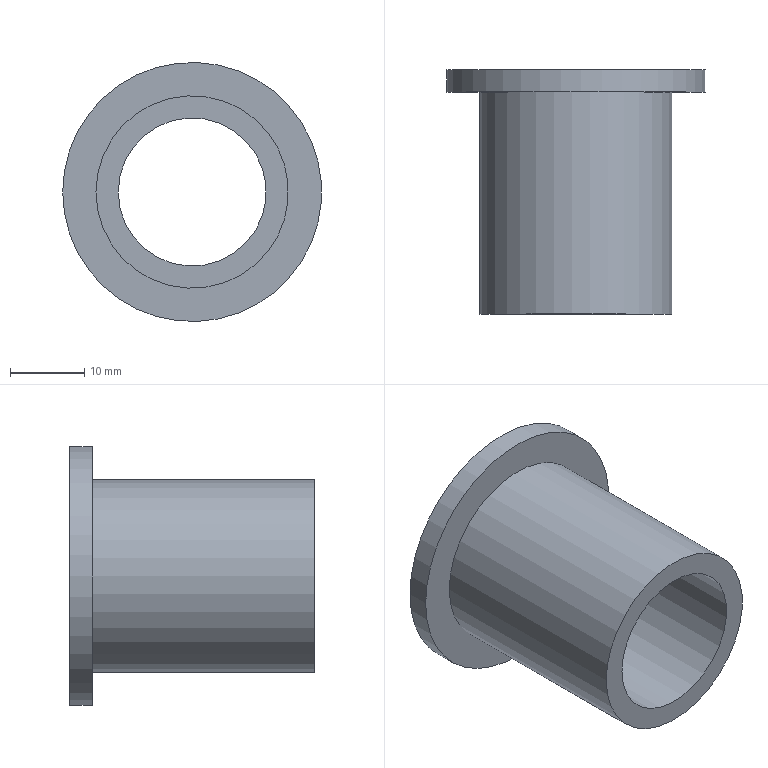Component | NX | BUSHING | 1 solid | 6 faces | box 35 x 33 x 35 mm | volume 8447 mm3 | cylinder 3 | plane 3 | commonest cylinder face diameters 26 x1 20 x1 35 x1
STEP:
#1=CARTESIAN_POINT('',(0.,0.,0.));
#2=DIRECTION('',(0.,0.,1.));
#3=DIRECTION('',(1.,0.,0.));
#4=AXIS2_PLACEMENT_3D('',#1,#2,#3);
#5=CARTESIAN_POINT('',(-13.,30.,66.));
#6=VERTEX_POINT('',#5);
#7=CARTESIAN_POINT('',(0.,30.,66.));
#8=DIRECTION('',(0.,1.,0.));
#9=DIRECTION('',(-1.,0.,0.));
#10=AXIS2_PLACEMENT_3D('',#7,#8,#9);
#11=CIRCLE('',#10,13.);
#12=CARTESIAN_POINT('',(0.,30.,66.));
#13=DIRECTION('',(0.,-1.,0.));
#14=DIRECTION('',(0.,0.,1.));
#15=AXIS2_PLACEMENT_3D('',#12,#13,#14);
#16=CYLINDRICAL_SURFACE('',#15,13.);
#17=CARTESIAN_POINT('',(7.854,0.));
#18=DIRECTION('',(-1.,0.));
#19=VECTOR('',#18,1.);
#20=LINE('',#17,#19);
#21=(GEOMETRIC_REPRESENTATION_CONTEXT(2)PARAMETRIC_REPRESENTATION_CONTEXT()REPRESENTATION_CONTEXT('',''));
#22=DEFINITIONAL_REPRESENTATION('',(#20),#21);
#23=PCURVE('',#16,#22);
#24=CARTESIAN_POINT('',(0.,30.,66.));
#25=DIRECTION('',(0.,1.,0.));
#26=DIRECTION('',(0.,0.,-1.));
#27=AXIS2_PLACEMENT_3D('',#24,#25,#26);
#28=PLANE('',#27);
#29=CARTESIAN_POINT('',(0.,0.));
#30=DIRECTION('',(0.,1.));
#31=AXIS2_PLACEMENT_2D('',#29,#30);
#32=CIRCLE('',#31,13.);
#33=(GEOMETRIC_REPRESENTATION_CONTEXT(2)PARAMETRIC_REPRESENTATION_CONTEXT()REPRESENTATION_CONTEXT('',''));
#34=DEFINITIONAL_REPRESENTATION('',(#32),#33);
#35=PCURVE('',#28,#34);
#36=SURFACE_CURVE('',#11,(#23,#35),.PCURVE_S1.);
#37=EDGE_CURVE('',#6,#6,#36,.T.);
#38=ORIENTED_EDGE('',*,*,#37,.F.);
#39=CARTESIAN_POINT('',(-13.,-0.,66.));
#40=VERTEX_POINT('',#39);
#41=CARTESIAN_POINT('',(-13.,30.,66.));
#42=CARTESIAN_POINT('',(-13.,-0.,66.));
#43=B_SPLINE_CURVE_WITH_KNOTS('',1,(#41,#42),.UNSPECIFIED.,.F.,.F.,(2,2),(0.,30.),.PIECEWISE_BEZIER_KNOTS.);
#44=CARTESIAN_POINT('',(7.854,0.));
#45=DIRECTION('',(0.,1.));
#46=VECTOR('',#45,1.);
#47=LINE('',#44,#46);
#48=(GEOMETRIC_REPRESENTATION_CONTEXT(2)PARAMETRIC_REPRESENTATION_CONTEXT()REPRESENTATION_CONTEXT('',''));
#49=DEFINITIONAL_REPRESENTATION('',(#47),#48);
#50=PCURVE('',#16,#49);
#51=CARTESIAN_POINT('',(1.571,0.));
#52=DIRECTION('',(0.,1.));
#53=VECTOR('',#52,1.);
#54=LINE('',#51,#53);
#55=(GEOMETRIC_REPRESENTATION_CONTEXT(2)PARAMETRIC_REPRESENTATION_CONTEXT()REPRESENTATION_CONTEXT('',''));
#56=DEFINITIONAL_REPRESENTATION('',(#54),#55);
#57=PCURVE('',#16,#56);
#58=SEAM_CURVE('',#43,(#50,#57),.PCURVE_S1.);
#59=EDGE_CURVE('',#6,#40,#58,.T.);
#60=ORIENTED_EDGE('',*,*,#59,.T.);
#61=CARTESIAN_POINT('',(0.,-0.,66.));
#62=DIRECTION('',(0.,1.,0.));
#63=DIRECTION('',(-1.,0.,0.));
#64=AXIS2_PLACEMENT_3D('',#61,#62,#63);
#65=CIRCLE('',#64,13.);
#66=CARTESIAN_POINT('',(7.854,30.));
#67=DIRECTION('',(-1.,0.));
#68=VECTOR('',#67,1.);
#69=LINE('',#66,#68);
#70=(GEOMETRIC_REPRESENTATION_CONTEXT(2)PARAMETRIC_REPRESENTATION_CONTEXT()REPRESENTATION_CONTEXT('',''));
#71=DEFINITIONAL_REPRESENTATION('',(#69),#70);
#72=PCURVE('',#16,#71);
#73=CARTESIAN_POINT('',(0.,-0.,66.));
#74=DIRECTION('',(0.,1.,0.));
#75=DIRECTION('',(0.,0.,-1.));
#76=AXIS2_PLACEMENT_3D('',#73,#74,#75);
#77=PLANE('',#76);
#78=CARTESIAN_POINT('',(0.,0.));
#79=DIRECTION('',(0.,1.));
#80=AXIS2_PLACEMENT_2D('',#78,#79);
#81=CIRCLE('',#80,13.);
#82=(GEOMETRIC_REPRESENTATION_CONTEXT(2)PARAMETRIC_REPRESENTATION_CONTEXT()REPRESENTATION_CONTEXT('',''));
#83=DEFINITIONAL_REPRESENTATION('',(#81),#82);
#84=PCURVE('',#77,#83);
#85=SURFACE_CURVE('',#65,(#72,#84),.PCURVE_S1.);
#86=EDGE_CURVE('',#40,#40,#85,.T.);
#87=ORIENTED_EDGE('',*,*,#86,.T.);
#88=ORIENTED_EDGE('',*,*,#59,.F.);
#89=EDGE_LOOP('',(#38,#60,#87,#88));
#90=FACE_BOUND('',#89,.T.);
#91=ADVANCED_FACE('',(#90),#16,.T.);
#92=CARTESIAN_POINT('',(-10.,-0.,66.));
#93=VERTEX_POINT('',#92);
#94=CARTESIAN_POINT('',(0.,-0.,66.));
#95=DIRECTION('',(0.,1.,0.));
#96=DIRECTION('',(-1.,0.,0.));
#97=AXIS2_PLACEMENT_3D('',#94,#95,#96);
#98=CIRCLE('',#97,10.);
#99=CARTESIAN_POINT('',(0.,30.,66.));
#100=DIRECTION('',(0.,-1.,0.));
#101=DIRECTION('',(0.,0.,1.));
#102=AXIS2_PLACEMENT_3D('',#99,#100,#101);
#103=CYLINDRICAL_SURFACE('',#102,10.);
#104=CARTESIAN_POINT('',(7.854,30.));
#105=DIRECTION('',(-1.,0.));
#106=VECTOR('',#105,1.);
#107=LINE('',#104,#106);
#108=(GEOMETRIC_REPRESENTATION_CONTEXT(2)PARAMETRIC_REPRESENTATION_CONTEXT()REPRESENTATION_CONTEXT('',''));
#109=DEFINITIONAL_REPRESENTATION('',(#107),#108);
#110=PCURVE('',#103,#109);
#111=CARTESIAN_POINT('',(0.,0.));
#112=DIRECTION('',(0.,1.));
#113=AXIS2_PLACEMENT_2D('',#111,#112);
#114=CIRCLE('',#113,10.);
#115=(GEOMETRIC_REPRESENTATION_CONTEXT(2)PARAMETRIC_REPRESENTATION_CONTEXT()REPRESENTATION_CONTEXT('',''));
#116=DEFINITIONAL_REPRESENTATION('',(#114),#115);
#117=PCURVE('',#77,#116);
#118=SURFACE_CURVE('',#98,(#110,#117),.PCURVE_S1.);
#119=EDGE_CURVE('',#93,#93,#118,.T.);
#120=ORIENTED_EDGE('',*,*,#119,.T.);
#121=CARTESIAN_POINT('',(-10.,33.,66.));
#122=VERTEX_POINT('',#121);
#123=CARTESIAN_POINT('',(-10.,33.,66.));
#124=CARTESIAN_POINT('',(-10.,0.,66.));
#125=B_SPLINE_CURVE_WITH_KNOTS('',1,(#123,#124),.UNSPECIFIED.,.F.,.F.,(2,2),(-3.,30.),.PIECEWISE_BEZIER_KNOTS.);
#126=CARTESIAN_POINT('',(1.571,0.));
#127=DIRECTION('',(0.,1.));
#128=VECTOR('',#127,1.);
#129=LINE('',#126,#128);
#130=(GEOMETRIC_REPRESENTATION_CONTEXT(2)PARAMETRIC_REPRESENTATION_CONTEXT()REPRESENTATION_CONTEXT('',''));
#131=DEFINITIONAL_REPRESENTATION('',(#129),#130);
#132=PCURVE('',#103,#131);
#133=CARTESIAN_POINT('',(7.854,0.));
#134=DIRECTION('',(0.,1.));
#135=VECTOR('',#134,1.);
#136=LINE('',#133,#135);
#137=(GEOMETRIC_REPRESENTATION_CONTEXT(2)PARAMETRIC_REPRESENTATION_CONTEXT()REPRESENTATION_CONTEXT('',''));
#138=DEFINITIONAL_REPRESENTATION('',(#136),#137);
#139=PCURVE('',#103,#138);
#140=SEAM_CURVE('',#125,(#132,#139),.PCURVE_S1.);
#141=EDGE_CURVE('',#122,#93,#140,.T.);
#142=ORIENTED_EDGE('',*,*,#141,.F.);
#143=CARTESIAN_POINT('',(0.,33.,66.));
#144=DIRECTION('',(0.,1.,0.));
#145=DIRECTION('',(-1.,0.,0.));
#146=AXIS2_PLACEMENT_3D('',#143,#144,#145);
#147=CIRCLE('',#146,10.);
#148=CARTESIAN_POINT('',(7.854,-3.));
#149=DIRECTION('',(-1.,0.));
#150=VECTOR('',#149,1.);
#151=LINE('',#148,#150);
#152=(GEOMETRIC_REPRESENTATION_CONTEXT(2)PARAMETRIC_REPRESENTATION_CONTEXT()REPRESENTATION_CONTEXT('',''));
#153=DEFINITIONAL_REPRESENTATION('',(#151),#152);
#154=PCURVE('',#103,#153);
#155=CARTESIAN_POINT('',(0.,33.,66.));
#156=DIRECTION('',(0.,1.,0.));
#157=DIRECTION('',(0.,0.,-1.));
#158=AXIS2_PLACEMENT_3D('',#155,#156,#157);
#159=PLANE('',#158);
#160=CARTESIAN_POINT('',(0.,0.));
#161=DIRECTION('',(0.,1.));
#162=AXIS2_PLACEMENT_2D('',#160,#161);
#163=CIRCLE('',#162,10.);
#164=(GEOMETRIC_REPRESENTATION_CONTEXT(2)PARAMETRIC_REPRESENTATION_CONTEXT()REPRESENTATION_CONTEXT('',''));
#165=DEFINITIONAL_REPRESENTATION('',(#163),#164);
#166=PCURVE('',#159,#165);
#167=SURFACE_CURVE('',#147,(#154,#166),.PCURVE_S1.);
#168=EDGE_CURVE('',#122,#122,#167,.T.);
#169=ORIENTED_EDGE('',*,*,#168,.F.);
#170=ORIENTED_EDGE('',*,*,#141,.T.);
#171=EDGE_LOOP('',(#120,#142,#169,#170));
#172=FACE_BOUND('',#171,.F.);
#173=ADVANCED_FACE('',(#172),#103,.F.);
#174=ORIENTED_EDGE('',*,*,#86,.F.);
#175=EDGE_LOOP('',(#174));
#176=FACE_BOUND('',#175,.T.);
#177=ORIENTED_EDGE('',*,*,#119,.T.);
#178=EDGE_LOOP('',(#177));
#179=FACE_BOUND('',#178,.T.);
#180=ADVANCED_FACE('',(#176,#179),#77,.F.);
#181=CARTESIAN_POINT('',(-17.5,30.,66.));
#182=VERTEX_POINT('',#181);
#183=CARTESIAN_POINT('',(0.,30.,66.));
#184=DIRECTION('',(0.,1.,0.));
#185=DIRECTION('',(-1.,0.,0.));
#186=AXIS2_PLACEMENT_3D('',#183,#184,#185);
#187=CIRCLE('',#186,17.5);
#188=CARTESIAN_POINT('',(0.,0.));
#189=DIRECTION('',(0.,1.));
#190=AXIS2_PLACEMENT_2D('',#188,#189);
#191=CIRCLE('',#190,17.5);
#192=(GEOMETRIC_REPRESENTATION_CONTEXT(2)PARAMETRIC_REPRESENTATION_CONTEXT()REPRESENTATION_CONTEXT('',''));
#193=DEFINITIONAL_REPRESENTATION('',(#191),#192);
#194=PCURVE('',#28,#193);
#195=CARTESIAN_POINT('',(0.,33.,66.));
#196=DIRECTION('',(0.,-1.,0.));
#197=DIRECTION('',(0.,0.,1.));
#198=AXIS2_PLACEMENT_3D('',#195,#196,#197);
#199=CYLINDRICAL_SURFACE('',#198,17.5);
#200=CARTESIAN_POINT('',(7.854,3.));
#201=DIRECTION('',(-1.,0.));
#202=VECTOR('',#201,1.);
#203=LINE('',#200,#202);
#204=(GEOMETRIC_REPRESENTATION_CONTEXT(2)PARAMETRIC_REPRESENTATION_CONTEXT()REPRESENTATION_CONTEXT('',''));
#205=DEFINITIONAL_REPRESENTATION('',(#203),#204);
#206=PCURVE('',#199,#205);
#207=SURFACE_CURVE('',#187,(#194,#206),.PCURVE_S1.);
#208=EDGE_CURVE('',#182,#182,#207,.T.);
#209=ORIENTED_EDGE('',*,*,#208,.F.);
#210=EDGE_LOOP('',(#209));
#211=FACE_BOUND('',#210,.T.);
#212=ORIENTED_EDGE('',*,*,#37,.T.);
#213=EDGE_LOOP('',(#212));
#214=FACE_BOUND('',#213,.T.);
#215=ADVANCED_FACE('',(#211,#214),#28,.F.);
#216=CARTESIAN_POINT('',(-17.5,33.,66.));
#217=VERTEX_POINT('',#216);
#218=CARTESIAN_POINT('',(0.,33.,66.));
#219=DIRECTION('',(0.,1.,0.));
#220=DIRECTION('',(-1.,0.,0.));
#221=AXIS2_PLACEMENT_3D('',#218,#219,#220);
#222=CIRCLE('',#221,17.5);
#223=CARTESIAN_POINT('',(7.854,0.));
#224=DIRECTION('',(-1.,0.));
#225=VECTOR('',#224,1.);
#226=LINE('',#223,#225);
#227=(GEOMETRIC_REPRESENTATION_CONTEXT(2)PARAMETRIC_REPRESENTATION_CONTEXT()REPRESENTATION_CONTEXT('',''));
#228=DEFINITIONAL_REPRESENTATION('',(#226),#227);
#229=PCURVE('',#199,#228);
#230=CARTESIAN_POINT('',(0.,0.));
#231=DIRECTION('',(0.,1.));
#232=AXIS2_PLACEMENT_2D('',#230,#231);
#233=CIRCLE('',#232,17.5);
#234=(GEOMETRIC_REPRESENTATION_CONTEXT(2)PARAMETRIC_REPRESENTATION_CONTEXT()REPRESENTATION_CONTEXT('',''));
#235=DEFINITIONAL_REPRESENTATION('',(#233),#234);
#236=PCURVE('',#159,#235);
#237=SURFACE_CURVE('',#222,(#229,#236),.PCURVE_S1.);
#238=EDGE_CURVE('',#217,#217,#237,.T.);
#239=ORIENTED_EDGE('',*,*,#238,.F.);
#240=CARTESIAN_POINT('',(-17.5,33.,66.));
#241=CARTESIAN_POINT('',(-17.5,30.,66.));
#242=B_SPLINE_CURVE_WITH_KNOTS('',1,(#240,#241),.UNSPECIFIED.,.F.,.F.,(2,2),(0.,3.),.PIECEWISE_BEZIER_KNOTS.);
#243=CARTESIAN_POINT('',(7.854,0.));
#244=DIRECTION('',(0.,1.));
#245=VECTOR('',#244,1.);
#246=LINE('',#243,#245);
#247=(GEOMETRIC_REPRESENTATION_CONTEXT(2)PARAMETRIC_REPRESENTATION_CONTEXT()REPRESENTATION_CONTEXT('',''));
#248=DEFINITIONAL_REPRESENTATION('',(#246),#247);
#249=PCURVE('',#199,#248);
#250=CARTESIAN_POINT('',(1.571,0.));
#251=DIRECTION('',(0.,1.));
#252=VECTOR('',#251,1.);
#253=LINE('',#250,#252);
#254=(GEOMETRIC_REPRESENTATION_CONTEXT(2)PARAMETRIC_REPRESENTATION_CONTEXT()REPRESENTATION_CONTEXT('',''));
#255=DEFINITIONAL_REPRESENTATION('',(#253),#254);
#256=PCURVE('',#199,#255);
#257=SEAM_CURVE('',#242,(#249,#256),.PCURVE_S1.);
#258=EDGE_CURVE('',#217,#182,#257,.T.);
#259=ORIENTED_EDGE('',*,*,#258,.T.);
#260=ORIENTED_EDGE('',*,*,#208,.T.);
#261=ORIENTED_EDGE('',*,*,#258,.F.);
#262=EDGE_LOOP('',(#239,#259,#260,#261));
#263=FACE_BOUND('',#262,.T.);
#264=ADVANCED_FACE('',(#263),#199,.T.);
#265=ORIENTED_EDGE('',*,*,#238,.T.);
#266=EDGE_LOOP('',(#265));
#267=FACE_BOUND('',#266,.T.);
#268=ORIENTED_EDGE('',*,*,#168,.F.);
#269=EDGE_LOOP('',(#268));
#270=FACE_BOUND('',#269,.T.);
#271=ADVANCED_FACE('',(#267,#270),#159,.T.);
#272=CLOSED_SHELL('',(#91,#173,#180,#215,#264,#271));
#273=MANIFOLD_SOLID_BREP('',#272);
#274=(LENGTH_UNIT()NAMED_UNIT(*)SI_UNIT(.MILLI.,.METRE.));
#275=UNCERTAINTY_MEASURE_WITH_UNIT(LENGTH_MEASURE(0.00001),#274,'','');
#276=(NAMED_UNIT(*)PLANE_ANGLE_UNIT()SI_UNIT($,.RADIAN.));
#277=(NAMED_UNIT(*)SI_UNIT($,.STERADIAN.)SOLID_ANGLE_UNIT());
#278=(GEOMETRIC_REPRESENTATION_CONTEXT(3)GLOBAL_UNCERTAINTY_ASSIGNED_CONTEXT((#275))GLOBAL_UNIT_ASSIGNED_CONTEXT((#274,#276,#277))REPRESENTATION_CONTEXT('',''));
#279=ADVANCED_BREP_SHAPE_REPRESENTATION('',(#4,#273),#278);